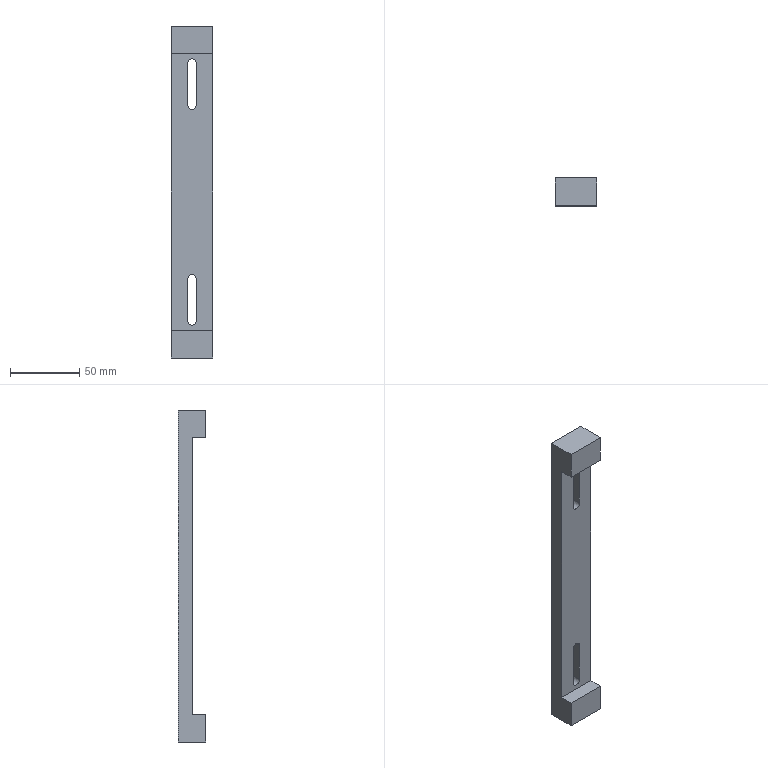Component | SolidWorks | CS021-A10-A022-2 | 1 solid | 18 faces | box 30 x 20 x 240 mm | volume 80545 mm3 | plane 14 | cylinder 4 | commonest cylinder face diameters 6.5 x4 | material AL6061
build123d program:
from build123d import *

# Parameters (mm, degrees)
BOSS_EXTRUDE1_DEPTH = 15
CUT_EXTRUDE1_REACH  = 124.577


with BuildPart() as part:
    # Sketch1 → Boss-Extrude1 (new, symmetric)
    with BuildSketch(Plane.XY):
        Polygon((-120, 0), (-120, 20), (120, 20), (120, 0), (100, 0), (100, 9.8), (-100, 9.8), (-100, 0), align=None)
    extrude(amount=BOSS_EXTRUDE1_DEPTH, both=True)

    # Sketch2 → Cut-Extrude1 (cut, up to next)
    with BuildSketch(Plane(origin=(0, 20, 0), x_dir=(1, 0, 0), z_dir=(0, 1, 0)), mode=Mode.PRIVATE) as cut_extrude1_sk1:
        with BuildLine():
            Line((63, 3.25), (93, 3.25))
            ThreePointArc((93, 3.25), (96.25, 0), (93, -3.25))
            Line((93, -3.25), (63, -3.25))
            ThreePointArc((63, -3.25), (59.75, 0), (63, 3.25))
        make_face()
    cut_extrude1_tool1 = extrude(cut_extrude1_sk1.sketch, amount=-CUT_EXTRUDE1_REACH, mode=Mode.PRIVATE) & part.part
    # Sketch2 → Cut-Extrude1 (cut, up to next)
    with BuildSketch(Plane(origin=(0, 20, 0), x_dir=(1, 0, 0), z_dir=(0, 1, 0)), mode=Mode.PRIVATE) as cut_extrude1_sk2:
        with BuildLine():
            Line((-63, 3.25), (-93, 3.25))
            ThreePointArc((-93, 3.25), (-96.25, 0), (-93, -3.25))
            Line((-93, -3.25), (-63, -3.25))
            ThreePointArc((-63, -3.25), (-59.75, 0), (-63, 3.25))
        make_face()
    cut_extrude1_tool2 = extrude(cut_extrude1_sk2.sketch, amount=-CUT_EXTRUDE1_REACH, mode=Mode.PRIVATE) & part.part
    add(cut_extrude1_tool1.solids().sort_by_distance((78, 20, 0))[0], mode=Mode.SUBTRACT)
    add(cut_extrude1_tool2.solids().sort_by_distance((-78, 20, 0))[0], mode=Mode.SUBTRACT)


solid = part.part

# Placed as in the assembly
solid = solid.moved(Location((30.949, 15.017, 0), (0, 90, 0)))
STEP:
#1=COLOUR_RGB('',0.7922,0.8196,0.9333);
#2=FILL_AREA_STYLE_COLOUR('',#1);
#3=FILL_AREA_STYLE('',(#2));
#4=SURFACE_STYLE_FILL_AREA(#3);
#5=SURFACE_SIDE_STYLE('',(#4));
#6=SURFACE_STYLE_USAGE(.BOTH.,#5);
#7=PRESENTATION_STYLE_ASSIGNMENT((#6));
#8=CARTESIAN_POINT('',(1.809,0.5912,-4.724));
#9=VERTEX_POINT('',#8);
#10=CARTESIAN_POINT('',(1.809,0.5912,-3.937));
#11=VERTEX_POINT('',#10);
#12=CARTESIAN_POINT('',(1.809,0.5912,-3.937));
#13=DIRECTION('',(0.,-0.,1.));
#14=VECTOR('',#13,39.37);
#15=LINE('',#12,#14);
#16=EDGE_CURVE('',#9,#11,#15,.T.);
#17=ORIENTED_EDGE('',*,*,#16,.T.);
#18=CARTESIAN_POINT('',(0.6279,0.5912,-3.937));
#19=VERTEX_POINT('',#18);
#20=CARTESIAN_POINT('',(0.6279,0.5912,-3.937));
#21=DIRECTION('',(1.,0.,-0.));
#22=VECTOR('',#21,39.37);
#23=LINE('',#20,#22);
#24=EDGE_CURVE('',#19,#11,#23,.T.);
#25=ORIENTED_EDGE('',*,*,#24,.F.);
#26=CARTESIAN_POINT('',(0.6279,0.5912,-4.724));
#27=VERTEX_POINT('',#26);
#28=CARTESIAN_POINT('',(0.6279,0.5912,-3.937));
#29=DIRECTION('',(0.,-0.,1.));
#30=VECTOR('',#29,39.37);
#31=LINE('',#28,#30);
#32=EDGE_CURVE('',#27,#19,#31,.T.);
#33=ORIENTED_EDGE('',*,*,#32,.F.);
#34=CARTESIAN_POINT('',(0.6279,0.5912,-4.724));
#35=DIRECTION('',(1.,0.,-0.));
#36=VECTOR('',#35,39.37);
#37=LINE('',#34,#36);
#38=EDGE_CURVE('',#27,#9,#37,.T.);
#39=ORIENTED_EDGE('',*,*,#38,.T.);
#40=EDGE_LOOP('',(#17,#25,#33,#39));
#41=FACE_OUTER_BOUND('',#40,.T.);
#42=CARTESIAN_POINT('',(0.6279,0.5912,-3.937));
#43=DIRECTION('',(-0.,1.,0.));
#44=DIRECTION('',(-0.,0.,-1.));
#45=AXIS2_PLACEMENT_3D('',#42,#43,#44);
#46=PLANE('',#45);
#47=ADVANCED_FACE('',(#41),#46,.F.);
#48=CARTESIAN_POINT('',(1.809,0.977,-3.937));
#49=VERTEX_POINT('',#48);
#50=CARTESIAN_POINT('',(1.809,0.977,-3.937));
#51=DIRECTION('',(-0.,1.,0.));
#52=VECTOR('',#51,39.37);
#53=LINE('',#50,#52);
#54=EDGE_CURVE('',#11,#49,#53,.T.);
#55=ORIENTED_EDGE('',*,*,#54,.T.);
#56=CARTESIAN_POINT('',(0.6279,0.977,-3.937));
#57=VERTEX_POINT('',#56);
#58=CARTESIAN_POINT('',(0.6279,0.977,-3.937));
#59=DIRECTION('',(1.,0.,-0.));
#60=VECTOR('',#59,39.37);
#61=LINE('',#58,#60);
#62=EDGE_CURVE('',#57,#49,#61,.T.);
#63=ORIENTED_EDGE('',*,*,#62,.F.);
#64=CARTESIAN_POINT('',(0.6279,0.977,-3.937));
#65=DIRECTION('',(-0.,1.,0.));
#66=VECTOR('',#65,39.37);
#67=LINE('',#64,#66);
#68=EDGE_CURVE('',#19,#57,#67,.T.);
#69=ORIENTED_EDGE('',*,*,#68,.F.);
#70=ORIENTED_EDGE('',*,*,#24,.T.);
#71=EDGE_LOOP('',(#55,#63,#69,#70));
#72=FACE_OUTER_BOUND('',#71,.T.);
#73=CARTESIAN_POINT('',(0.6279,0.977,-3.937));
#74=DIRECTION('',(-0.,0.,-1.));
#75=DIRECTION('',(-1.,0.,0.));
#76=AXIS2_PLACEMENT_3D('',#73,#74,#75);
#77=PLANE('',#76);
#78=ADVANCED_FACE('',(#72),#77,.F.);
#79=CARTESIAN_POINT('',(1.09,0.977,-2.48));
#80=VERTEX_POINT('',#79);
#81=CARTESIAN_POINT('',(1.09,0.977,-3.661));
#82=VERTEX_POINT('',#81);
#83=CARTESIAN_POINT('',(1.09,0.977,-2.48));
#84=DIRECTION('',(-0.,-0.,-1.));
#85=VECTOR('',#84,39.37);
#86=LINE('',#83,#85);
#87=EDGE_CURVE('',#80,#82,#86,.T.);
#88=ORIENTED_EDGE('',*,*,#87,.F.);
#89=CARTESIAN_POINT('',(1.346,0.977,-2.48));
#90=VERTEX_POINT('',#89);
#91=CARTESIAN_POINT('',(1.218,0.977,-2.48));
#92=DIRECTION('',(0.,-1.,0.));
#93=DIRECTION('',(0.,0.,-1.));
#94=AXIS2_PLACEMENT_3D('',#91,#92,#93);
#95=CIRCLE('',#94,0.128);
#96=EDGE_CURVE('',#90,#80,#95,.T.);
#97=ORIENTED_EDGE('',*,*,#96,.F.);
#98=CARTESIAN_POINT('',(1.346,0.977,-3.661));
#99=VERTEX_POINT('',#98);
#100=CARTESIAN_POINT('',(1.346,0.977,-2.48));
#101=DIRECTION('',(0.,0.,1.));
#102=VECTOR('',#101,39.37);
#103=LINE('',#100,#102);
#104=EDGE_CURVE('',#99,#90,#103,.T.);
#105=ORIENTED_EDGE('',*,*,#104,.F.);
#106=CARTESIAN_POINT('',(1.218,0.977,-3.661));
#107=DIRECTION('',(0.,-1.,0.));
#108=DIRECTION('',(0.,0.,-1.));
#109=AXIS2_PLACEMENT_3D('',#106,#107,#108);
#110=CIRCLE('',#109,0.128);
#111=EDGE_CURVE('',#82,#99,#110,.T.);
#112=ORIENTED_EDGE('',*,*,#111,.F.);
#113=EDGE_LOOP('',(#88,#97,#105,#112));
#114=FACE_BOUND('',#113,.T.);
#115=CARTESIAN_POINT('',(1.346,0.977,2.48));
#116=VERTEX_POINT('',#115);
#117=CARTESIAN_POINT('',(1.346,0.977,3.661));
#118=VERTEX_POINT('',#117);
#119=CARTESIAN_POINT('',(1.346,0.977,2.48));
#120=DIRECTION('',(0.,0.,1.));
#121=VECTOR('',#120,39.37);
#122=LINE('',#119,#121);
#123=EDGE_CURVE('',#116,#118,#122,.T.);
#124=ORIENTED_EDGE('',*,*,#123,.F.);
#125=CARTESIAN_POINT('',(1.09,0.977,2.48));
#126=VERTEX_POINT('',#125);
#127=CARTESIAN_POINT('',(1.218,0.977,2.48));
#128=DIRECTION('',(0.,-1.,0.));
#129=DIRECTION('',(0.,0.,-1.));
#130=AXIS2_PLACEMENT_3D('',#127,#128,#129);
#131=CIRCLE('',#130,0.128);
#132=EDGE_CURVE('',#126,#116,#131,.T.);
#133=ORIENTED_EDGE('',*,*,#132,.F.);
#134=CARTESIAN_POINT('',(1.09,0.977,3.661));
#135=VERTEX_POINT('',#134);
#136=CARTESIAN_POINT('',(1.09,0.977,2.48));
#137=DIRECTION('',(-0.,-0.,-1.));
#138=VECTOR('',#137,39.37);
#139=LINE('',#136,#138);
#140=EDGE_CURVE('',#135,#126,#139,.T.);
#141=ORIENTED_EDGE('',*,*,#140,.F.);
#142=CARTESIAN_POINT('',(1.218,0.977,3.661));
#143=DIRECTION('',(0.,-1.,0.));
#144=DIRECTION('',(0.,0.,-1.));
#145=AXIS2_PLACEMENT_3D('',#142,#143,#144);
#146=CIRCLE('',#145,0.128);
#147=EDGE_CURVE('',#118,#135,#146,.T.);
#148=ORIENTED_EDGE('',*,*,#147,.F.);
#149=EDGE_LOOP('',(#124,#133,#141,#148));
#150=FACE_BOUND('',#149,.T.);
#151=CARTESIAN_POINT('',(1.809,0.977,3.937));
#152=VERTEX_POINT('',#151);
#153=CARTESIAN_POINT('',(1.809,0.977,3.937));
#154=DIRECTION('',(0.,0.,1.));
#155=VECTOR('',#154,39.37);
#156=LINE('',#153,#155);
#157=EDGE_CURVE('',#49,#152,#156,.T.);
#158=ORIENTED_EDGE('',*,*,#157,.T.);
#159=CARTESIAN_POINT('',(0.6279,0.977,3.937));
#160=VERTEX_POINT('',#159);
#161=CARTESIAN_POINT('',(0.6279,0.977,3.937));
#162=DIRECTION('',(1.,0.,-0.));
#163=VECTOR('',#162,39.37);
#164=LINE('',#161,#163);
#165=EDGE_CURVE('',#160,#152,#164,.T.);
#166=ORIENTED_EDGE('',*,*,#165,.F.);
#167=CARTESIAN_POINT('',(0.6279,0.977,3.937));
#168=DIRECTION('',(0.,0.,1.));
#169=VECTOR('',#168,39.37);
#170=LINE('',#167,#169);
#171=EDGE_CURVE('',#57,#160,#170,.T.);
#172=ORIENTED_EDGE('',*,*,#171,.F.);
#173=ORIENTED_EDGE('',*,*,#62,.T.);
#174=EDGE_LOOP('',(#158,#166,#172,#173));
#175=FACE_OUTER_BOUND('',#174,.T.);
#176=CARTESIAN_POINT('',(0.6279,0.977,3.937));
#177=DIRECTION('',(-0.,1.,-0.));
#178=DIRECTION('',(-0.,-0.,-1.));
#179=AXIS2_PLACEMENT_3D('',#176,#177,#178);
#180=PLANE('',#179);
#181=ADVANCED_FACE('',(#114,#150,#175),#180,.F.);
#182=CARTESIAN_POINT('',(1.809,0.5912,3.937));
#183=VERTEX_POINT('',#182);
#184=CARTESIAN_POINT('',(1.809,0.977,3.937));
#185=DIRECTION('',(0.,-1.,-0.));
#186=VECTOR('',#185,39.37);
#187=LINE('',#184,#186);
#188=EDGE_CURVE('',#152,#183,#187,.T.);
#189=ORIENTED_EDGE('',*,*,#188,.T.);
#190=CARTESIAN_POINT('',(0.6279,0.5912,3.937));
#191=VERTEX_POINT('',#190);
#192=CARTESIAN_POINT('',(0.6279,0.5912,3.937));
#193=DIRECTION('',(1.,0.,-0.));
#194=VECTOR('',#193,39.37);
#195=LINE('',#192,#194);
#196=EDGE_CURVE('',#191,#183,#195,.T.);
#197=ORIENTED_EDGE('',*,*,#196,.F.);
#198=CARTESIAN_POINT('',(0.6279,0.977,3.937));
#199=DIRECTION('',(0.,-1.,-0.));
#200=VECTOR('',#199,39.37);
#201=LINE('',#198,#200);
#202=EDGE_CURVE('',#160,#191,#201,.T.);
#203=ORIENTED_EDGE('',*,*,#202,.F.);
#204=ORIENTED_EDGE('',*,*,#165,.T.);
#205=EDGE_LOOP('',(#189,#197,#203,#204));
#206=FACE_OUTER_BOUND('',#205,.T.);
#207=CARTESIAN_POINT('',(0.6279,0.977,3.937));
#208=DIRECTION('',(0.,-0.,1.));
#209=DIRECTION('',(1.,0.,-0.));
#210=AXIS2_PLACEMENT_3D('',#207,#208,#209);
#211=PLANE('',#210);
#212=ADVANCED_FACE('',(#206),#211,.F.);
#213=CARTESIAN_POINT('',(1.809,0.5912,4.724));
#214=VERTEX_POINT('',#213);
#215=CARTESIAN_POINT('',(1.809,0.5912,3.937));
#216=DIRECTION('',(0.,0.,1.));
#217=VECTOR('',#216,39.37);
#218=LINE('',#215,#217);
#219=EDGE_CURVE('',#183,#214,#218,.T.);
#220=ORIENTED_EDGE('',*,*,#219,.T.);
#221=CARTESIAN_POINT('',(0.6279,0.5912,4.724));
#222=VERTEX_POINT('',#221);
#223=CARTESIAN_POINT('',(0.6279,0.5912,4.724));
#224=DIRECTION('',(1.,0.,-0.));
#225=VECTOR('',#224,39.37);
#226=LINE('',#223,#225);
#227=EDGE_CURVE('',#222,#214,#226,.T.);
#228=ORIENTED_EDGE('',*,*,#227,.F.);
#229=CARTESIAN_POINT('',(0.6279,0.5912,3.937));
#230=DIRECTION('',(0.,0.,1.));
#231=VECTOR('',#230,39.37);
#232=LINE('',#229,#231);
#233=EDGE_CURVE('',#191,#222,#232,.T.);
#234=ORIENTED_EDGE('',*,*,#233,.F.);
#235=ORIENTED_EDGE('',*,*,#196,.T.);
#236=EDGE_LOOP('',(#220,#228,#234,#235));
#237=FACE_OUTER_BOUND('',#236,.T.);
#238=CARTESIAN_POINT('',(0.6279,0.5912,3.937));
#239=DIRECTION('',(-0.,1.,-0.));
#240=DIRECTION('',(-0.,-0.,-1.));
#241=AXIS2_PLACEMENT_3D('',#238,#239,#240);
#242=PLANE('',#241);
#243=ADVANCED_FACE('',(#237),#242,.F.);
#244=CARTESIAN_POINT('',(1.809,1.379,4.724));
#245=VERTEX_POINT('',#244);
#246=CARTESIAN_POINT('',(1.809,0.5912,4.724));
#247=DIRECTION('',(-0.,1.,0.));
#248=VECTOR('',#247,39.37);
#249=LINE('',#246,#248);
#250=EDGE_CURVE('',#214,#245,#249,.T.);
#251=ORIENTED_EDGE('',*,*,#250,.T.);
#252=CARTESIAN_POINT('',(0.6279,1.379,4.724));
#253=VERTEX_POINT('',#252);
#254=CARTESIAN_POINT('',(0.6279,1.379,4.724));
#255=DIRECTION('',(1.,0.,-0.));
#256=VECTOR('',#255,39.37);
#257=LINE('',#254,#256);
#258=EDGE_CURVE('',#253,#245,#257,.T.);
#259=ORIENTED_EDGE('',*,*,#258,.F.);
#260=CARTESIAN_POINT('',(0.6279,0.5912,4.724));
#261=DIRECTION('',(-0.,1.,0.));
#262=VECTOR('',#261,39.37);
#263=LINE('',#260,#262);
#264=EDGE_CURVE('',#222,#253,#263,.T.);
#265=ORIENTED_EDGE('',*,*,#264,.F.);
#266=ORIENTED_EDGE('',*,*,#227,.T.);
#267=EDGE_LOOP('',(#251,#259,#265,#266));
#268=FACE_OUTER_BOUND('',#267,.T.);
#269=CARTESIAN_POINT('',(0.6279,0.5912,4.724));
#270=DIRECTION('',(-0.,0.,-1.));
#271=DIRECTION('',(-1.,0.,0.));
#272=AXIS2_PLACEMENT_3D('',#269,#270,#271);
#273=PLANE('',#272);
#274=ADVANCED_FACE('',(#268),#273,.F.);
#275=CARTESIAN_POINT('',(1.346,1.379,-2.48));
#276=VERTEX_POINT('',#275);
#277=CARTESIAN_POINT('',(1.346,1.379,-3.661));
#278=VERTEX_POINT('',#277);
#279=CARTESIAN_POINT('',(1.346,1.379,-2.48));
#280=DIRECTION('',(-0.,0.,-1.));
#281=VECTOR('',#280,39.37);
#282=LINE('',#279,#281);
#283=EDGE_CURVE('',#276,#278,#282,.T.);
#284=ORIENTED_EDGE('',*,*,#283,.F.);
#285=CARTESIAN_POINT('',(1.09,1.379,-2.48));
#286=VERTEX_POINT('',#285);
#287=CARTESIAN_POINT('',(1.218,1.379,-2.48));
#288=DIRECTION('',(-0.,1.,0.));
#289=DIRECTION('',(1.,0.,0.));
#290=AXIS2_PLACEMENT_3D('',#287,#288,#289);
#291=CIRCLE('',#290,0.128);
#292=EDGE_CURVE('',#286,#276,#291,.T.);
#293=ORIENTED_EDGE('',*,*,#292,.F.);
#294=CARTESIAN_POINT('',(1.09,1.379,-3.661));
#295=VERTEX_POINT('',#294);
#296=CARTESIAN_POINT('',(1.09,1.379,-2.48));
#297=DIRECTION('',(0.,-0.,1.));
#298=VECTOR('',#297,39.37);
#299=LINE('',#296,#298);
#300=EDGE_CURVE('',#295,#286,#299,.T.);
#301=ORIENTED_EDGE('',*,*,#300,.F.);
#302=CARTESIAN_POINT('',(1.218,1.379,-3.661));
#303=DIRECTION('',(-0.,1.,0.));
#304=DIRECTION('',(1.,0.,0.));
#305=AXIS2_PLACEMENT_3D('',#302,#303,#304);
#306=CIRCLE('',#305,0.128);
#307=EDGE_CURVE('',#278,#295,#306,.T.);
#308=ORIENTED_EDGE('',*,*,#307,.F.);
#309=EDGE_LOOP('',(#284,#293,#301,#308));
#310=FACE_BOUND('',#309,.T.);
#311=CARTESIAN_POINT('',(1.09,1.379,2.48));
#312=VERTEX_POINT('',#311);
#313=CARTESIAN_POINT('',(1.09,1.379,3.661));
#314=VERTEX_POINT('',#313);
#315=CARTESIAN_POINT('',(1.09,1.379,2.48));
#316=DIRECTION('',(0.,-0.,1.));
#317=VECTOR('',#316,39.37);
#318=LINE('',#315,#317);
#319=EDGE_CURVE('',#312,#314,#318,.T.);
#320=ORIENTED_EDGE('',*,*,#319,.F.);
#321=CARTESIAN_POINT('',(1.346,1.379,2.48));
#322=VERTEX_POINT('',#321);
#323=CARTESIAN_POINT('',(1.218,1.379,2.48));
#324=DIRECTION('',(-0.,1.,0.));
#325=DIRECTION('',(-1.,0.,0.));
#326=AXIS2_PLACEMENT_3D('',#323,#324,#325);
#327=CIRCLE('',#326,0.128);
#328=EDGE_CURVE('',#322,#312,#327,.T.);
#329=ORIENTED_EDGE('',*,*,#328,.F.);
#330=CARTESIAN_POINT('',(1.346,1.379,3.661));
#331=VERTEX_POINT('',#330);
#332=CARTESIAN_POINT('',(1.346,1.379,2.48));
#333=DIRECTION('',(-0.,0.,-1.));
#334=VECTOR('',#333,39.37);
#335=LINE('',#332,#334);
#336=EDGE_CURVE('',#331,#322,#335,.T.);
#337=ORIENTED_EDGE('',*,*,#336,.F.);
#338=CARTESIAN_POINT('',(1.218,1.379,3.661));
#339=DIRECTION('',(-0.,1.,0.));
#340=DIRECTION('',(-1.,0.,0.));
#341=AXIS2_PLACEMENT_3D('',#338,#339,#340);
#342=CIRCLE('',#341,0.128);
#343=EDGE_CURVE('',#314,#331,#342,.T.);
#344=ORIENTED_EDGE('',*,*,#343,.F.);
#345=EDGE_LOOP('',(#320,#329,#337,#344));
#346=FACE_BOUND('',#345,.T.);
#347=CARTESIAN_POINT('',(1.809,1.379,-4.724));
#348=VERTEX_POINT('',#347);
#349=CARTESIAN_POINT('',(1.809,1.379,-4.724));
#350=DIRECTION('',(-0.,0.,-1.));
#351=VECTOR('',#350,39.37);
#352=LINE('',#349,#351);
#353=EDGE_CURVE('',#245,#348,#352,.T.);
#354=ORIENTED_EDGE('',*,*,#353,.T.);
#355=CARTESIAN_POINT('',(0.6279,1.379,-4.724));
#356=VERTEX_POINT('',#355);
#357=CARTESIAN_POINT('',(0.6279,1.379,-4.724));
#358=DIRECTION('',(1.,0.,-0.));
#359=VECTOR('',#358,39.37);
#360=LINE('',#357,#359);
#361=EDGE_CURVE('',#356,#348,#360,.T.);
#362=ORIENTED_EDGE('',*,*,#361,.F.);
#363=CARTESIAN_POINT('',(0.6279,1.379,-4.724));
#364=DIRECTION('',(-0.,0.,-1.));
#365=VECTOR('',#364,39.37);
#366=LINE('',#363,#365);
#367=EDGE_CURVE('',#253,#356,#366,.T.);
#368=ORIENTED_EDGE('',*,*,#367,.F.);
#369=ORIENTED_EDGE('',*,*,#258,.T.);
#370=EDGE_LOOP('',(#354,#362,#368,#369));
#371=FACE_OUTER_BOUND('',#370,.T.);
#372=CARTESIAN_POINT('',(0.6279,1.379,-4.724));
#373=DIRECTION('',(-0.,-1.,-0.));
#374=DIRECTION('',(1.,0.,-0.));
#375=AXIS2_PLACEMENT_3D('',#372,#373,#374);
#376=PLANE('',#375);
#377=ADVANCED_FACE('',(#310,#346,#371),#376,.F.);
#378=CARTESIAN_POINT('',(1.809,0.5912,-4.724));
#379=DIRECTION('',(0.,-1.,-0.));
#380=VECTOR('',#379,39.37);
#381=LINE('',#378,#380);
#382=EDGE_CURVE('',#348,#9,#381,.T.);
#383=ORIENTED_EDGE('',*,*,#382,.T.);
#384=ORIENTED_EDGE('',*,*,#38,.F.);
#385=CARTESIAN_POINT('',(0.6279,0.5912,-4.724));
#386=DIRECTION('',(0.,-1.,-0.));
#387=VECTOR('',#386,39.37);
#388=LINE('',#385,#387);
#389=EDGE_CURVE('',#356,#27,#388,.T.);
#390=ORIENTED_EDGE('',*,*,#389,.F.);
#391=ORIENTED_EDGE('',*,*,#361,.T.);
#392=EDGE_LOOP('',(#383,#384,#390,#391));
#393=FACE_OUTER_BOUND('',#392,.T.);
#394=CARTESIAN_POINT('',(0.6279,0.5912,-4.724));
#395=DIRECTION('',(0.,-0.,1.));
#396=DIRECTION('',(1.,0.,-0.));
#397=AXIS2_PLACEMENT_3D('',#394,#395,#396);
#398=PLANE('',#397);
#399=ADVANCED_FACE('',(#393),#398,.F.);
#400=ORIENTED_EDGE('',*,*,#32,.T.);
#401=ORIENTED_EDGE('',*,*,#68,.T.);
#402=ORIENTED_EDGE('',*,*,#171,.T.);
#403=ORIENTED_EDGE('',*,*,#202,.T.);
#404=ORIENTED_EDGE('',*,*,#233,.T.);
#405=ORIENTED_EDGE('',*,*,#264,.T.);
#406=ORIENTED_EDGE('',*,*,#367,.T.);
#407=ORIENTED_EDGE('',*,*,#389,.T.);
#408=EDGE_LOOP('',(#400,#401,#402,#403,#404,#405,#406,#407));
#409=FACE_OUTER_BOUND('',#408,.T.);
#410=CARTESIAN_POINT('',(0.6279,0.5912,-0.));
#411=DIRECTION('',(1.,0.,-0.));
#412=DIRECTION('',(-0.,0.,-1.));
#413=AXIS2_PLACEMENT_3D('',#410,#411,#412);
#414=PLANE('',#413);
#415=ADVANCED_FACE('',(#409),#414,.F.);
#416=ORIENTED_EDGE('',*,*,#16,.F.);
#417=ORIENTED_EDGE('',*,*,#382,.F.);
#418=ORIENTED_EDGE('',*,*,#353,.F.);
#419=ORIENTED_EDGE('',*,*,#250,.F.);
#420=ORIENTED_EDGE('',*,*,#219,.F.);
#421=ORIENTED_EDGE('',*,*,#188,.F.);
#422=ORIENTED_EDGE('',*,*,#157,.F.);
#423=ORIENTED_EDGE('',*,*,#54,.F.);
#424=EDGE_LOOP('',(#416,#417,#418,#419,#420,#421,#422,#423));
#425=FACE_OUTER_BOUND('',#424,.T.);
#426=CARTESIAN_POINT('',(1.809,0.5912,-0.));
#427=DIRECTION('',(1.,0.,-0.));
#428=DIRECTION('',(-0.,0.,-1.));
#429=AXIS2_PLACEMENT_3D('',#426,#427,#428);
#430=PLANE('',#429);
#431=ADVANCED_FACE('',(#425),#430,.T.);
#432=ORIENTED_EDGE('',*,*,#132,.T.);
#433=CARTESIAN_POINT('',(1.346,0.5912,2.48));
#434=DIRECTION('',(-0.,1.,0.));
#435=VECTOR('',#434,39.37);
#436=LINE('',#433,#435);
#437=EDGE_CURVE('',#116,#322,#436,.T.);
#438=ORIENTED_EDGE('',*,*,#437,.T.);
#439=ORIENTED_EDGE('',*,*,#328,.T.);
#440=CARTESIAN_POINT('',(1.09,0.5912,2.48));
#441=DIRECTION('',(-0.,1.,0.));
#442=VECTOR('',#441,39.37);
#443=LINE('',#440,#442);
#444=EDGE_CURVE('',#126,#312,#443,.T.);
#445=ORIENTED_EDGE('',*,*,#444,.F.);
#446=EDGE_LOOP('',(#432,#438,#439,#445));
#447=FACE_OUTER_BOUND('',#446,.T.);
#448=CARTESIAN_POINT('',(1.218,0.5912,2.48));
#449=DIRECTION('',(-0.,1.,0.));
#450=DIRECTION('',(-1.,0.,0.));
#451=AXIS2_PLACEMENT_3D('',#448,#449,#450);
#452=CYLINDRICAL_SURFACE('',#451,0.128);
#453=ADVANCED_FACE('',(#447),#452,.F.);
#454=ORIENTED_EDGE('',*,*,#123,.T.);
#455=CARTESIAN_POINT('',(1.346,0.5912,3.661));
#456=DIRECTION('',(-0.,1.,0.));
#457=VECTOR('',#456,39.37);
#458=LINE('',#455,#457);
#459=EDGE_CURVE('',#118,#331,#458,.T.);
#460=ORIENTED_EDGE('',*,*,#459,.T.);
#461=ORIENTED_EDGE('',*,*,#336,.T.);
#462=ORIENTED_EDGE('',*,*,#437,.F.);
#463=EDGE_LOOP('',(#454,#460,#461,#462));
#464=FACE_OUTER_BOUND('',#463,.T.);
#465=CARTESIAN_POINT('',(1.346,0.5912,2.48));
#466=DIRECTION('',(1.,-0.,-0.));
#467=DIRECTION('',(-0.,0.,-1.));
#468=AXIS2_PLACEMENT_3D('',#465,#466,#467);
#469=PLANE('',#468);
#470=ADVANCED_FACE('',(#464),#469,.F.);
#471=ORIENTED_EDGE('',*,*,#147,.T.);
#472=CARTESIAN_POINT('',(1.09,0.5912,3.661));
#473=DIRECTION('',(-0.,1.,0.));
#474=VECTOR('',#473,39.37);
#475=LINE('',#472,#474);
#476=EDGE_CURVE('',#135,#314,#475,.T.);
#477=ORIENTED_EDGE('',*,*,#476,.T.);
#478=ORIENTED_EDGE('',*,*,#343,.T.);
#479=ORIENTED_EDGE('',*,*,#459,.F.);
#480=EDGE_LOOP('',(#471,#477,#478,#479));
#481=FACE_OUTER_BOUND('',#480,.T.);
#482=CARTESIAN_POINT('',(1.218,0.5912,3.661));
#483=DIRECTION('',(-0.,1.,0.));
#484=DIRECTION('',(-1.,0.,0.));
#485=AXIS2_PLACEMENT_3D('',#482,#483,#484);
#486=CYLINDRICAL_SURFACE('',#485,0.128);
#487=ADVANCED_FACE('',(#481),#486,.F.);
#488=ORIENTED_EDGE('',*,*,#140,.T.);
#489=ORIENTED_EDGE('',*,*,#444,.T.);
#490=ORIENTED_EDGE('',*,*,#319,.T.);
#491=ORIENTED_EDGE('',*,*,#476,.F.);
#492=EDGE_LOOP('',(#488,#489,#490,#491));
#493=FACE_OUTER_BOUND('',#492,.T.);
#494=CARTESIAN_POINT('',(1.09,0.5912,2.48));
#495=DIRECTION('',(-1.,-0.,0.));
#496=DIRECTION('',(0.,-0.,1.));
#497=AXIS2_PLACEMENT_3D('',#494,#495,#496);
#498=PLANE('',#497);
#499=ADVANCED_FACE('',(#493),#498,.F.);
#500=ORIENTED_EDGE('',*,*,#96,.T.);
#501=CARTESIAN_POINT('',(1.09,0.5912,-2.48));
#502=DIRECTION('',(-0.,1.,0.));
#503=VECTOR('',#502,39.37);
#504=LINE('',#501,#503);
#505=EDGE_CURVE('',#80,#286,#504,.T.);
#506=ORIENTED_EDGE('',*,*,#505,.T.);
#507=ORIENTED_EDGE('',*,*,#292,.T.);
#508=CARTESIAN_POINT('',(1.346,0.5912,-2.48));
#509=DIRECTION('',(-0.,1.,0.));
#510=VECTOR('',#509,39.37);
#511=LINE('',#508,#510);
#512=EDGE_CURVE('',#90,#276,#511,.T.);
#513=ORIENTED_EDGE('',*,*,#512,.F.);
#514=EDGE_LOOP('',(#500,#506,#507,#513));
#515=FACE_OUTER_BOUND('',#514,.T.);
#516=CARTESIAN_POINT('',(1.218,0.5912,-2.48));
#517=DIRECTION('',(-0.,1.,0.));
#518=DIRECTION('',(-1.,0.,0.));
#519=AXIS2_PLACEMENT_3D('',#516,#517,#518);
#520=CYLINDRICAL_SURFACE('',#519,0.128);
#521=ADVANCED_FACE('',(#515),#520,.F.);
#522=ORIENTED_EDGE('',*,*,#87,.T.);
#523=CARTESIAN_POINT('',(1.09,0.5912,-3.661));
#524=DIRECTION('',(-0.,1.,0.));
#525=VECTOR('',#524,39.37);
#526=LINE('',#523,#525);
#527=EDGE_CURVE('',#82,#295,#526,.T.);
#528=ORIENTED_EDGE('',*,*,#527,.T.);
#529=ORIENTED_EDGE('',*,*,#300,.T.);
#530=ORIENTED_EDGE('',*,*,#505,.F.);
#531=EDGE_LOOP('',(#522,#528,#529,#530));
#532=FACE_OUTER_BOUND('',#531,.T.);
#533=CARTESIAN_POINT('',(1.09,0.5912,-2.48));
#534=DIRECTION('',(-1.,0.,0.));
#535=DIRECTION('',(0.,-0.,1.));
#536=AXIS2_PLACEMENT_3D('',#533,#534,#535);
#537=PLANE('',#536);
#538=ADVANCED_FACE('',(#532),#537,.F.);
#539=ORIENTED_EDGE('',*,*,#111,.T.);
#540=CARTESIAN_POINT('',(1.346,0.5912,-3.661));
#541=DIRECTION('',(-0.,1.,0.));
#542=VECTOR('',#541,39.37);
#543=LINE('',#540,#542);
#544=EDGE_CURVE('',#99,#278,#543,.T.);
#545=ORIENTED_EDGE('',*,*,#544,.T.);
#546=ORIENTED_EDGE('',*,*,#307,.T.);
#547=ORIENTED_EDGE('',*,*,#527,.F.);
#548=EDGE_LOOP('',(#539,#545,#546,#547));
#549=FACE_OUTER_BOUND('',#548,.T.);
#550=CARTESIAN_POINT('',(1.218,0.5912,-3.661));
#551=DIRECTION('',(-0.,1.,0.));
#552=DIRECTION('',(-1.,0.,0.));
#553=AXIS2_PLACEMENT_3D('',#550,#551,#552);
#554=CYLINDRICAL_SURFACE('',#553,0.128);
#555=ADVANCED_FACE('',(#549),#554,.F.);
#556=ORIENTED_EDGE('',*,*,#104,.T.);
#557=ORIENTED_EDGE('',*,*,#512,.T.);
#558=ORIENTED_EDGE('',*,*,#283,.T.);
#559=ORIENTED_EDGE('',*,*,#544,.F.);
#560=EDGE_LOOP('',(#556,#557,#558,#559));
#561=FACE_OUTER_BOUND('',#560,.T.);
#562=CARTESIAN_POINT('',(1.346,0.5912,-2.48));
#563=DIRECTION('',(1.,0.,-0.));
#564=DIRECTION('',(-0.,0.,-1.));
#565=AXIS2_PLACEMENT_3D('',#562,#563,#564);
#566=PLANE('',#565);
#567=ADVANCED_FACE('',(#561),#566,.F.);
#568=CLOSED_SHELL('',(#47,#78,#181,#212,#243,#274,#377,#399,#415,#431,#453,#470,#487,#499,#521,#538,#555,#567));
#569=MANIFOLD_SOLID_BREP('',#568);
#570=STYLED_ITEM('',(#7),#569);
#571=PRESENTATION_LAYER_ASSIGNMENT('','',(#570));
#572=(LENGTH_UNIT()NAMED_UNIT(*)SI_UNIT($,.METRE.));
#573=LENGTH_MEASURE_WITH_UNIT(LENGTH_MEASURE(0.0254),#572);
#574=DIMENSIONAL_EXPONENTS(1.,0.,0.,0.,0.,0.,0.);
#575=(CONVERSION_BASED_UNIT('',#573)LENGTH_UNIT()NAMED_UNIT(#574));
#576=UNCERTAINTY_MEASURE_WITH_UNIT(LENGTH_MEASURE(0.00001),#575,'','');
#577=(NAMED_UNIT(*)PLANE_ANGLE_UNIT()SI_UNIT($,.RADIAN.));
#578=(NAMED_UNIT(*)SI_UNIT($,.STERADIAN.)SOLID_ANGLE_UNIT());
#579=(GEOMETRIC_REPRESENTATION_CONTEXT(3)GLOBAL_UNCERTAINTY_ASSIGNED_CONTEXT((#576))GLOBAL_UNIT_ASSIGNED_CONTEXT((#575,#577,#578))REPRESENTATION_CONTEXT('',''));
#580=MECHANICAL_DESIGN_GEOMETRIC_PRESENTATION_REPRESENTATION('',(#570),#579);
#581=CARTESIAN_POINT('',(0.,0.,0.));
#582=DIRECTION('',(0.,0.,1.));
#583=DIRECTION('',(1.,0.,0.));
#584=AXIS2_PLACEMENT_3D('',#581,#582,#583);
#585=(LENGTH_UNIT()NAMED_UNIT(*)SI_UNIT($,.METRE.));
#586=LENGTH_MEASURE_WITH_UNIT(LENGTH_MEASURE(0.0254),#585);
#587=DIMENSIONAL_EXPONENTS(1.,0.,0.,0.,0.,0.,0.);
#588=(CONVERSION_BASED_UNIT('',#586)LENGTH_UNIT()NAMED_UNIT(#587));
#589=UNCERTAINTY_MEASURE_WITH_UNIT(LENGTH_MEASURE(0.00001),#588,'','');
#590=(NAMED_UNIT(*)PLANE_ANGLE_UNIT()SI_UNIT($,.RADIAN.));
#591=(NAMED_UNIT(*)SI_UNIT($,.STERADIAN.)SOLID_ANGLE_UNIT());
#592=(GEOMETRIC_REPRESENTATION_CONTEXT(3)GLOBAL_UNCERTAINTY_ASSIGNED_CONTEXT((#589))GLOBAL_UNIT_ASSIGNED_CONTEXT((#588,#590,#591))REPRESENTATION_CONTEXT('',''));
#593=ADVANCED_BREP_SHAPE_REPRESENTATION('',(#569,#584),#592);